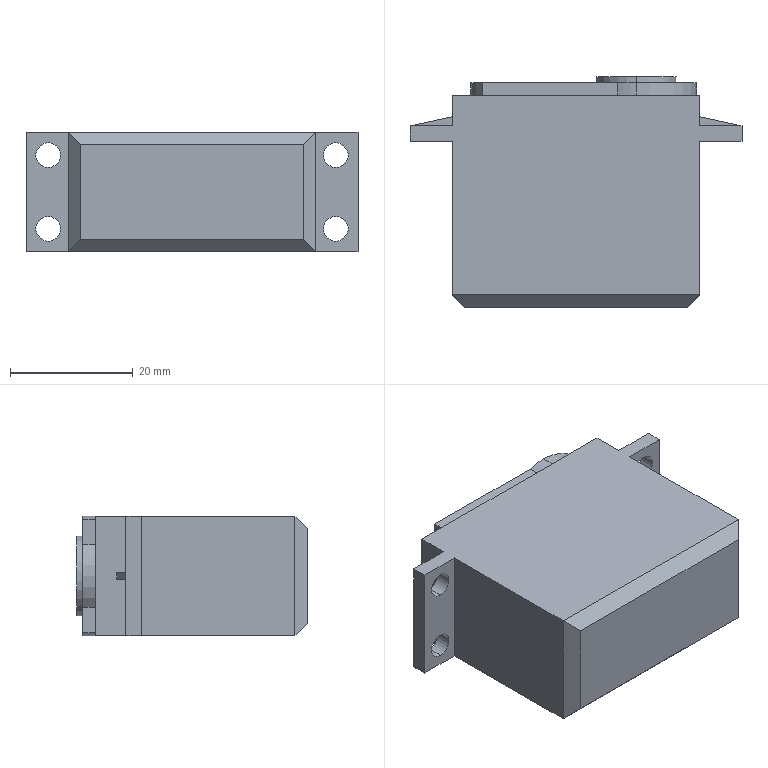Component | SolidWorks | MotorHousing-1 | 1 solid | 199 faces | volume 28611 mm3 | plane 114 | spline 69 | cylinder 16 | commonest cylinder face diameters 4 x8 19.5 x3 5.8 x2 13 x2 15 x1 | material CA